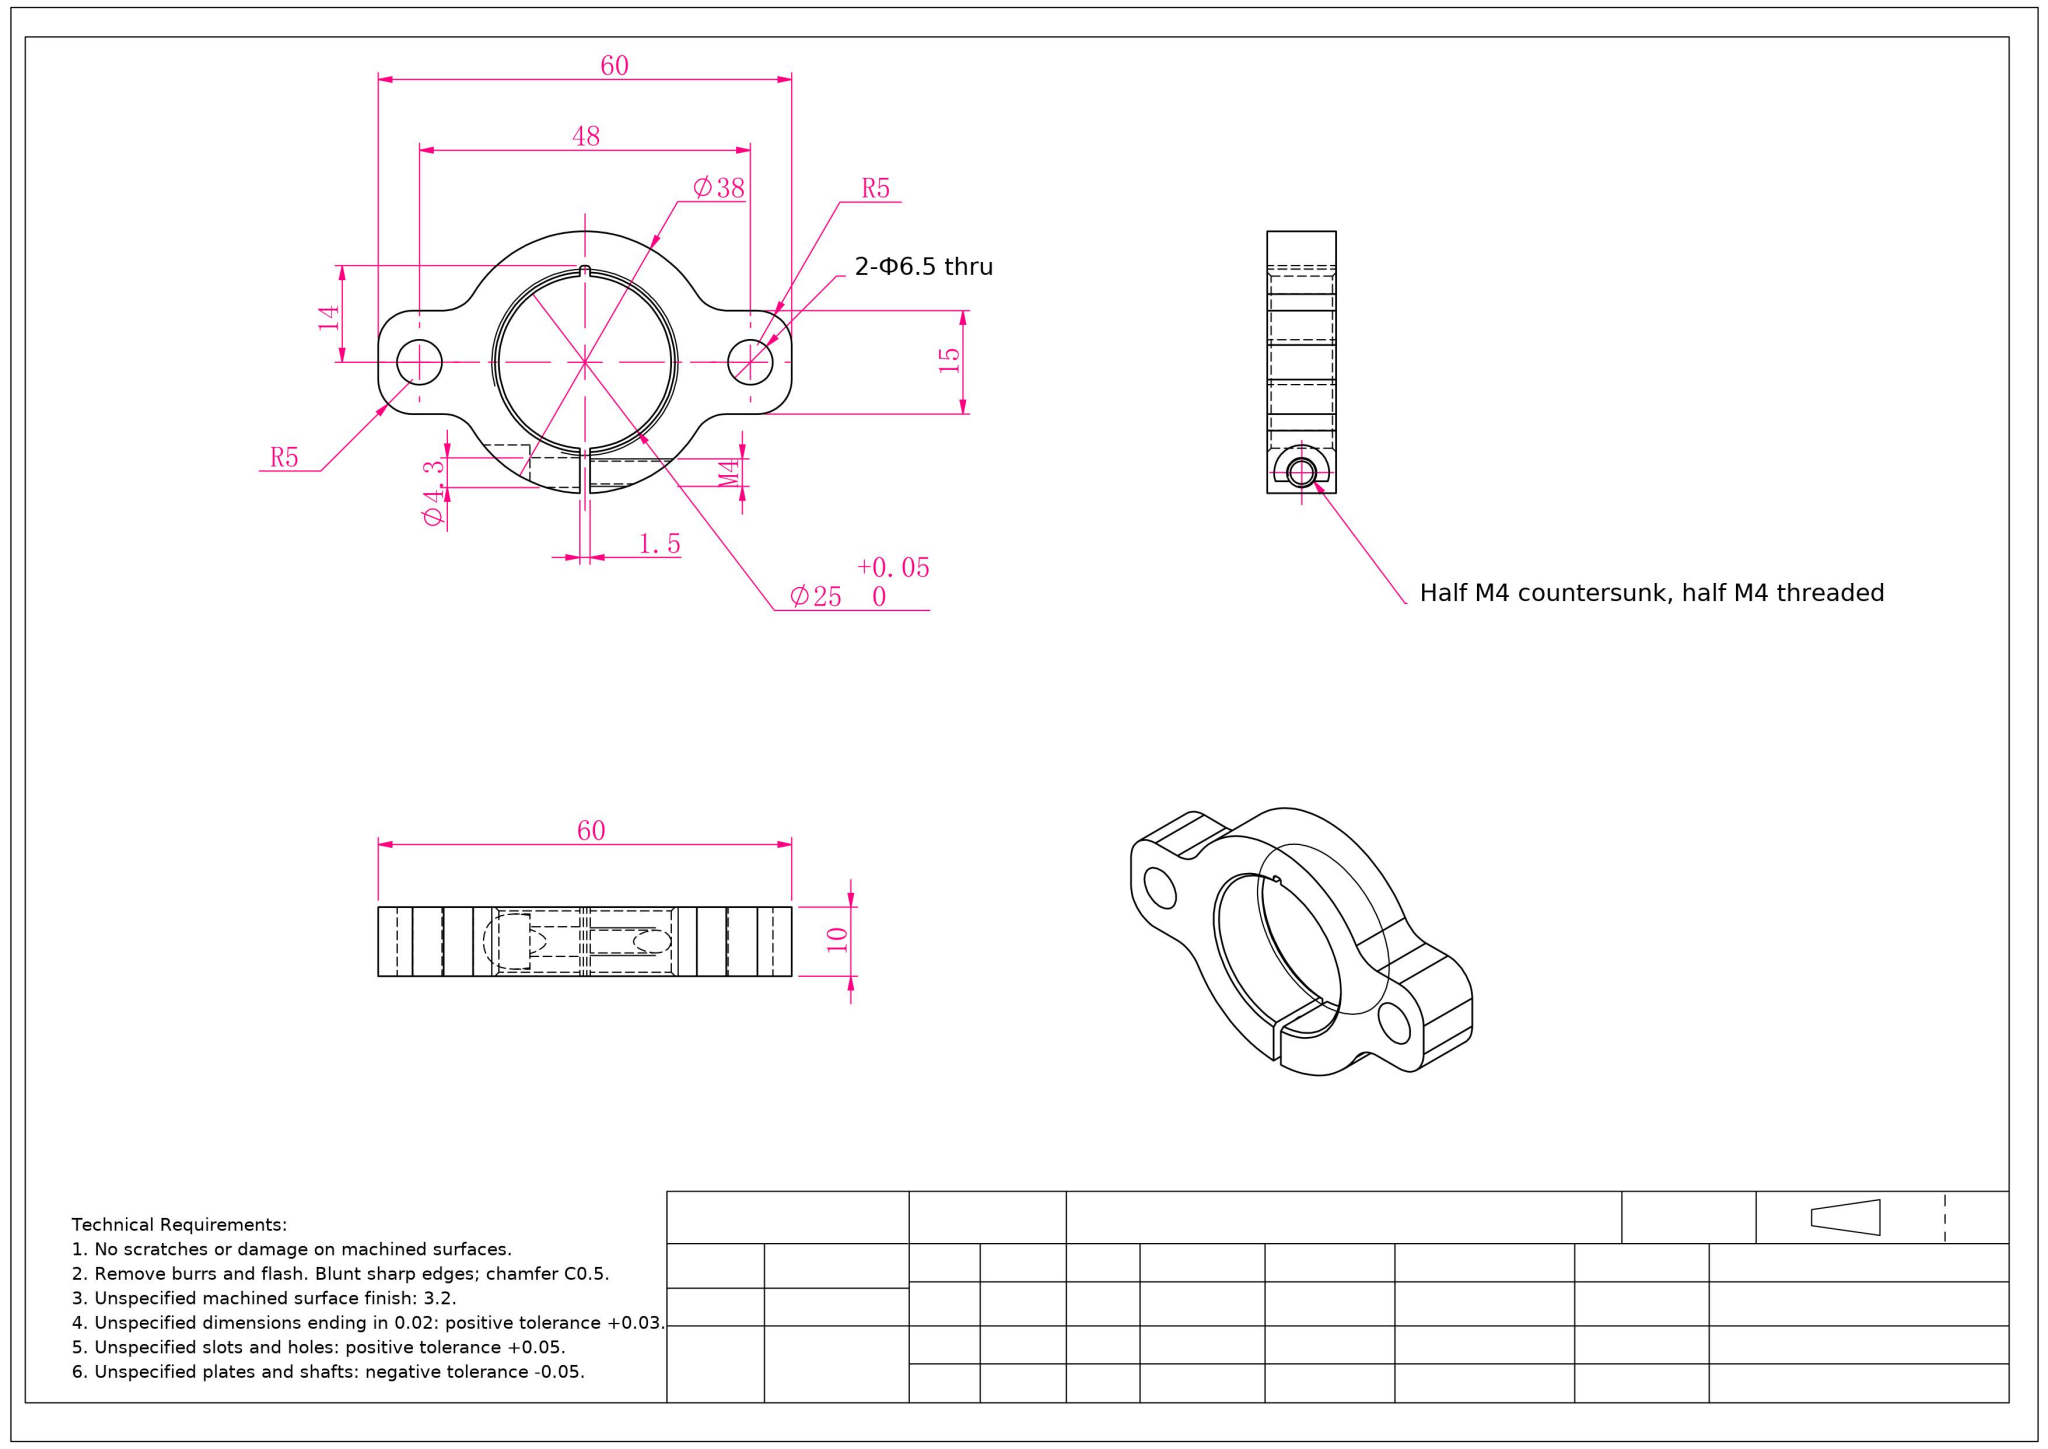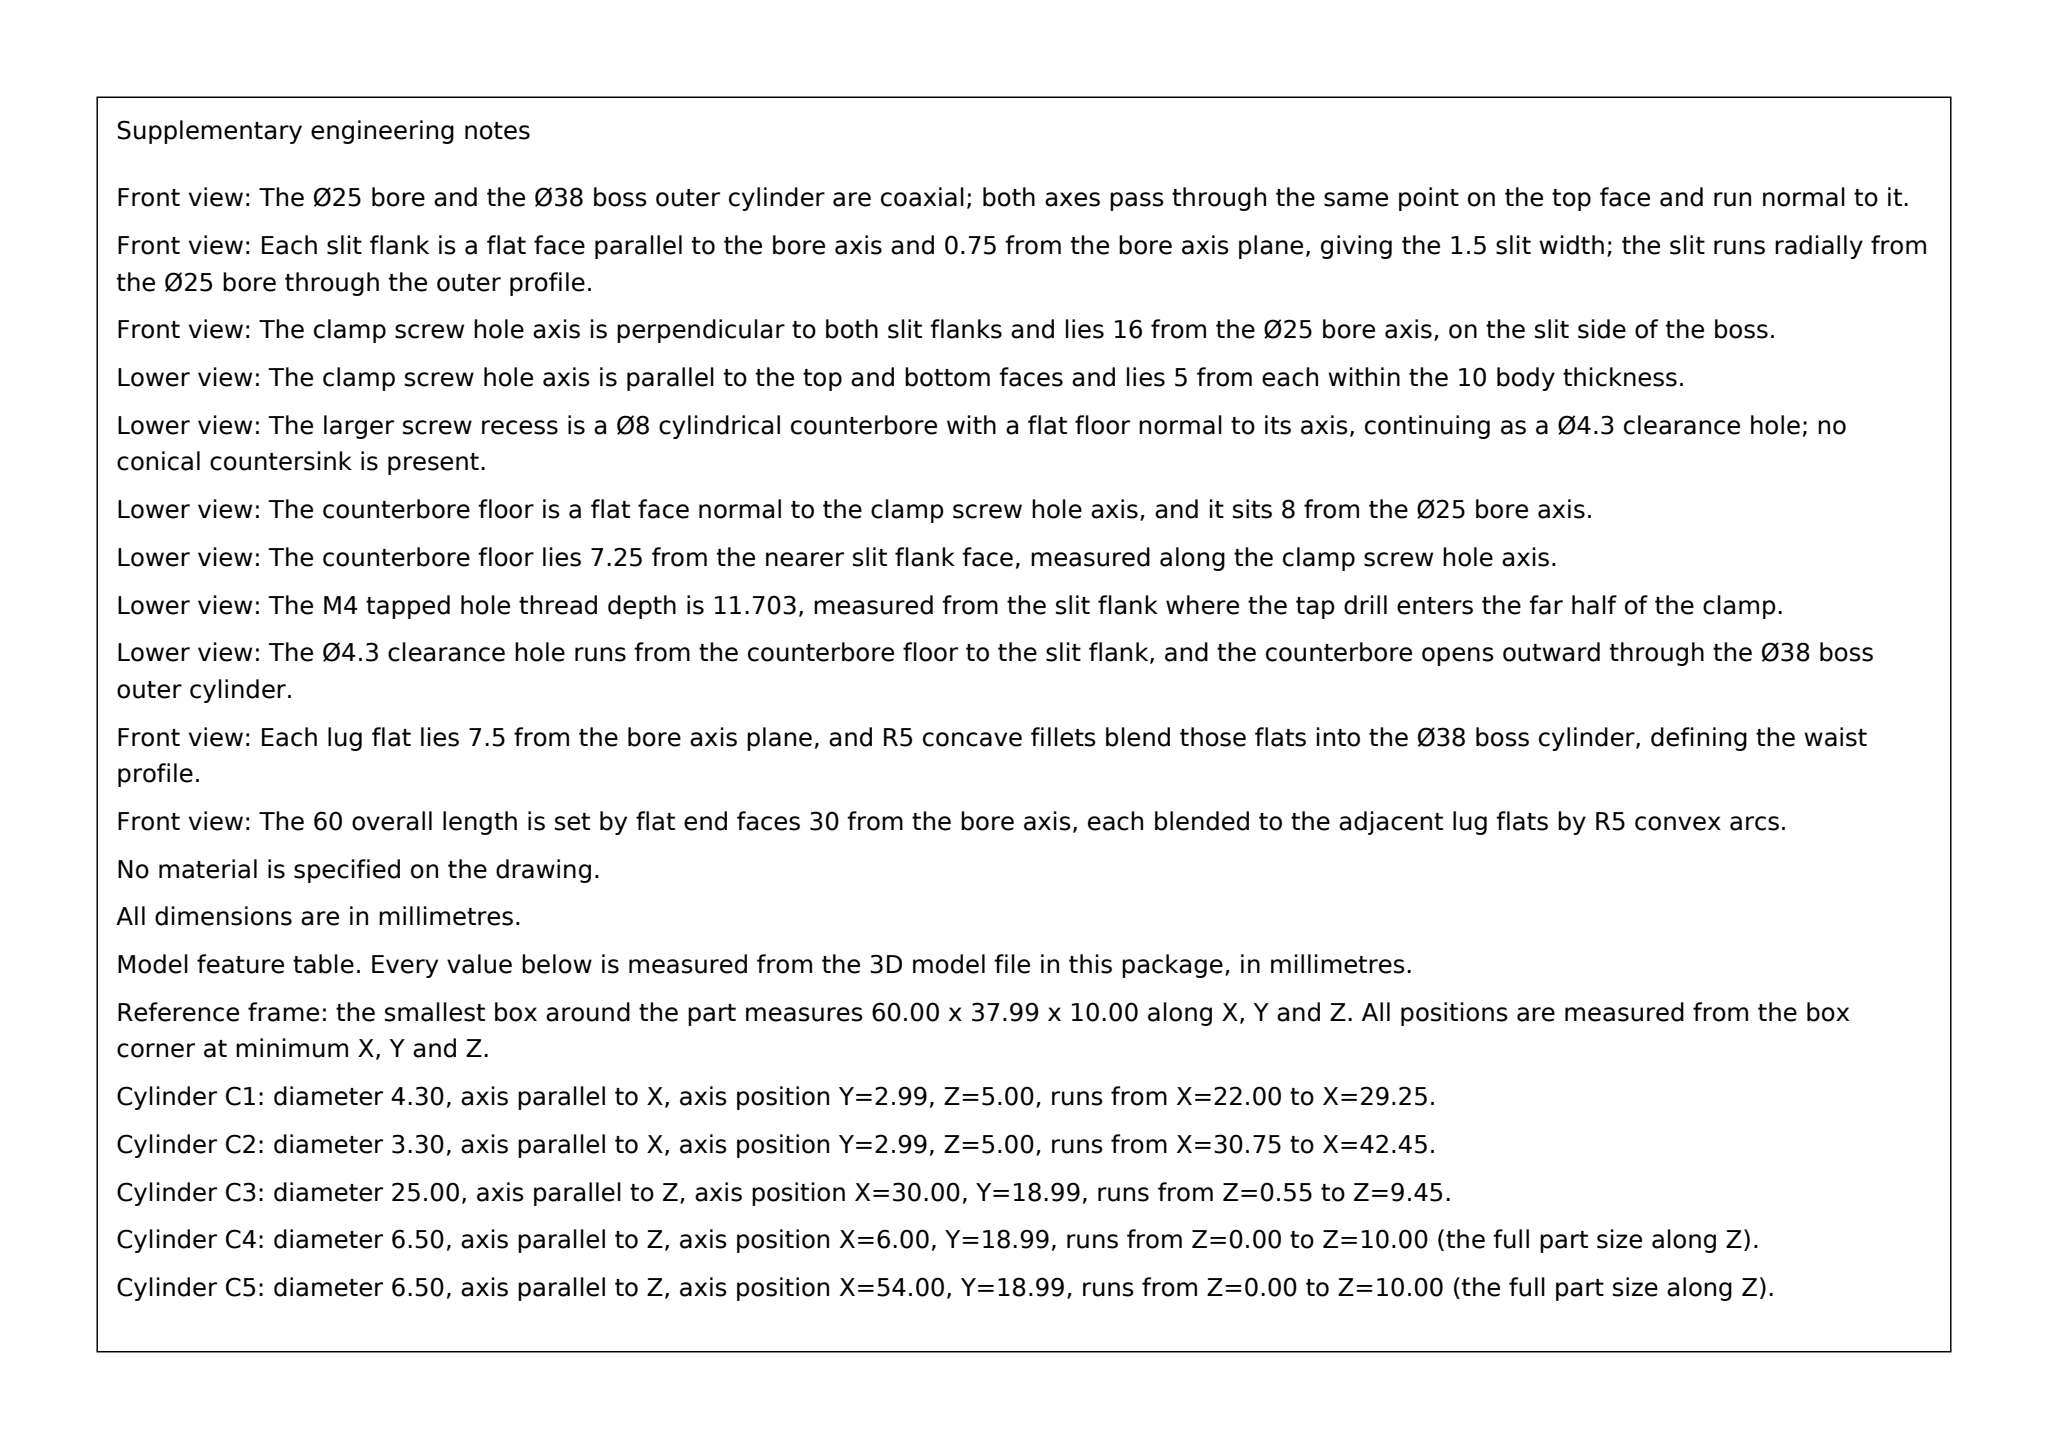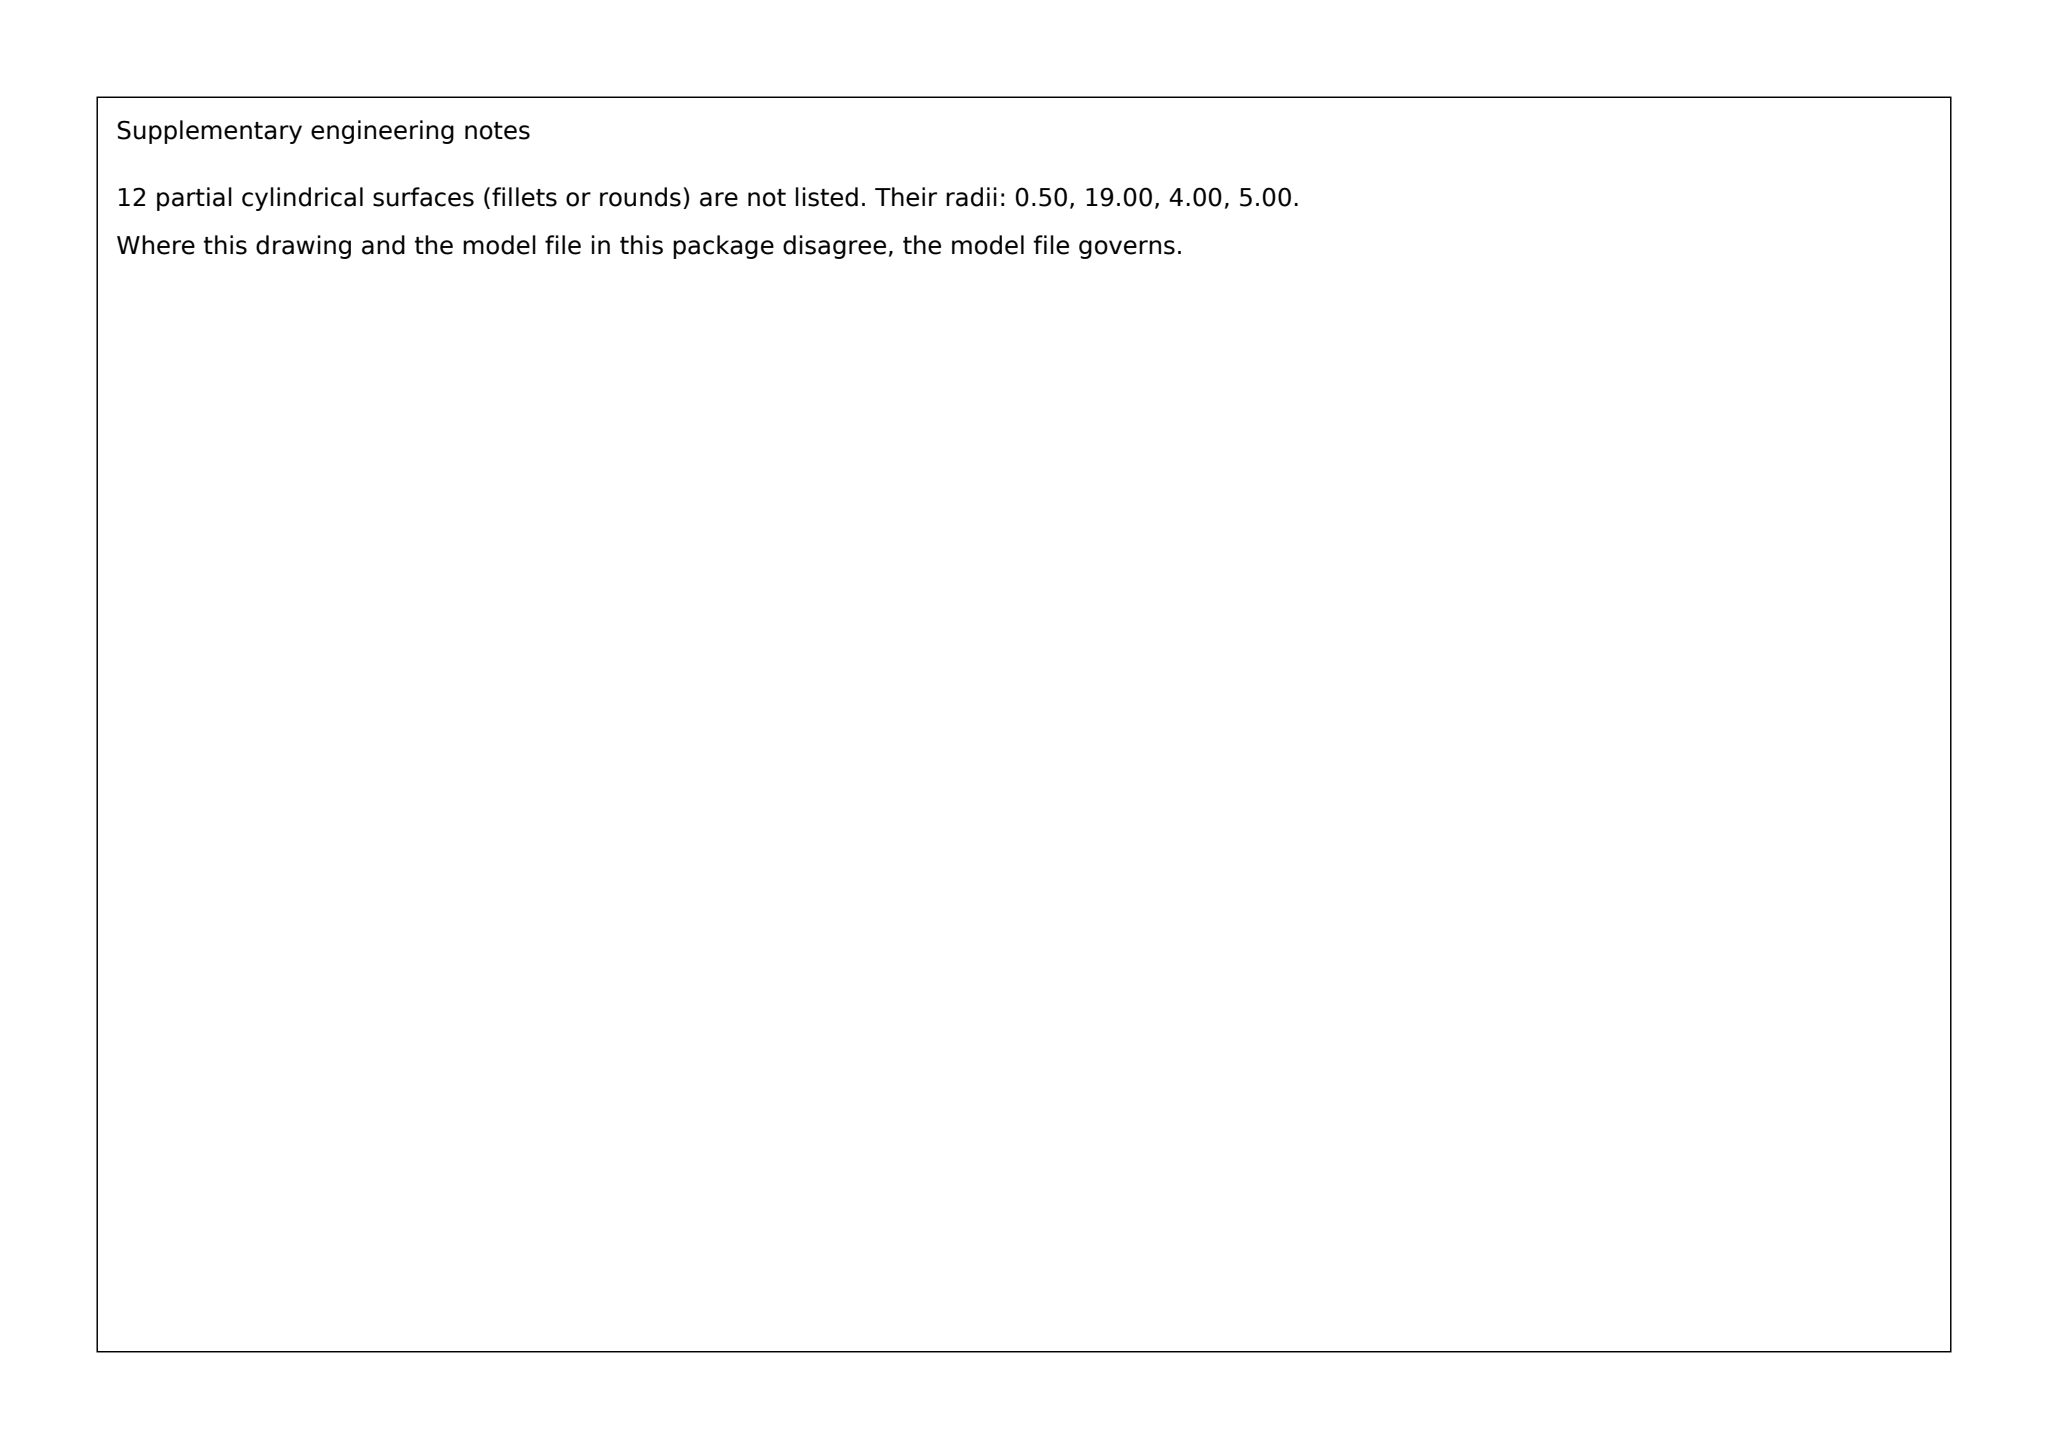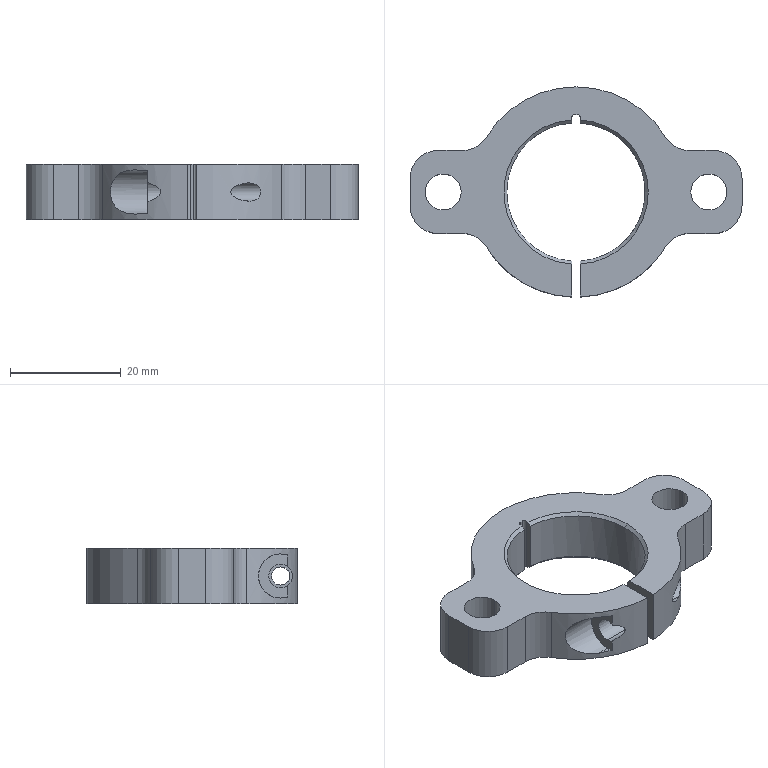Part | SolidWorks | mm | 1 solid | 47 faces | box 60 x 37.99 x 10 mm | volume 8615 mm3 | cylinder 27 | plane 14 | cone 6 | commonest cylinder face diameters 10 x8 6.5 x4 25 x3 8 x3 38 x3 4.3 x2 3.3 x2 1 x2
build123d program:
from build123d import *

# Parameters (mm, degrees)
SKETCH1_R                                       = 12.05
EXTRUDE1_DEPTH                                  = 10
SKETCH2_R                                       = 3.25
EXTRUDE2_DEPTH                                  = 37.892
EXTRUDE3_DEPTH                                  = 37.892
SKETCH4_W                                       = 1.65
SKETCH4_H                                       = 29.25
M4_HEX_SOCKET_HEAD_CAP_SCREW_HOLE_1_D           = 4.3
M4_HEX_SOCKET_HEAD_CAP_SCREW_HOLE_1_DEPTH       = 17.25
M4_HEX_SOCKET_HEAD_CAP_SCREW_HOLE_1_CBORE_D     = 8
M4_HEX_SOCKET_HEAD_CAP_SCREW_HOLE_1_CBORE_DEPTH = 10
FILLET1_R                                       = 5
CHAMFER1_SIZE                                   = 1
M27X2_0_TAPPED_HOLE1_D                          = 25


with BuildPart() as part:
    # Sketch1 → Extrude1 (new body)
    with BuildSketch(Plane.XY):
        with BuildLine():
            Line((-25, -7.5), (-17.457, -7.5))
            ThreePointArc((-17.457, -7.5), (0, -19), (17.457, -7.5))
            Line((17.457, -7.5), (25, -7.5))
            ThreePointArc((25, -7.5), (28.536, -6.036), (30, -2.5))
            Line((30, -2.5), (30, 2.5))
            ThreePointArc((30, 2.5), (28.536, 6.036), (25, 7.5))
            Line((25, 7.5), (17.457, 7.5))
            ThreePointArc((17.457, 7.5), (0, 19), (-17.457, 7.5))
            Line((-17.457, 7.5), (-25, 7.5))
            ThreePointArc((-25, 7.5), (-28.536, 6.036), (-30, 2.5))
            Line((-30, 2.5), (-30, -2.5))
            ThreePointArc((-30, -2.5), (-28.536, -6.036), (-25, -7.5))
        make_face()
        Circle(SKETCH1_R, mode=Mode.SUBTRACT)
    extrude(amount=EXTRUDE1_DEPTH)

    # Sketch2 → Extrude2 (cut, through all)
    with BuildSketch(Plane(origin=(0, 0, 0), x_dir=(-1, 0, 0), z_dir=(0, 0, -1))):
        with Locations((-24, 0)):
            Circle(SKETCH2_R)
        with Locations((24, 0)):
            Circle(SKETCH2_R)
    extrude(amount=-EXTRUDE2_DEPTH, mode=Mode.SUBTRACT)

    # Sketch3 → Extrude3 (cut, through all)
    with BuildSketch(Plane.XY.offset(10)):
        with BuildLine():
            Line((-0.25, 14), (0.25, 14))
            ThreePointArc((0.25, 14), (0.6036, 13.854), (0.75, 13.5))
            Line((0.75, 13.5), (0.75, -26.662))
            Line((0.75, -26.662), (-0.75, -26.662))
            Line((-0.75, -26.662), (-0.75, 13.5))
            ThreePointArc((-0.75, 13.5), (-0.6036, 13.854), (-0.25, 14))
        make_face()
    extrude(amount=-EXTRUDE3_DEPTH, mode=Mode.SUBTRACT)

    # Sketch4 → M4 Tapped Hole1 (revolve, cut)
    with BuildSketch(Plane(origin=(0.75, -16, 5), x_dir=(0, 0, 1), z_dir=(0, 1, 0))):
        with Locations((0.825, 14.625)):
            Rectangle(SKETCH4_W, SKETCH4_H)
    revolve(axis=Axis((-5.6, -16, 5), (1, 0, 0)), mode=Mode.SUBTRACT)

    # M4 Hex Socket Head Cap Screw Hole 1
    with Locations(Plane(origin=(-18, 0, 0), x_dir=(0, 0, -1), z_dir=(-1, 0, 0))):
        with Locations((-5, 16)):
            CounterBoreHole(M4_HEX_SOCKET_HEAD_CAP_SCREW_HOLE_1_D / 2, M4_HEX_SOCKET_HEAD_CAP_SCREW_HOLE_1_CBORE_D / 2, M4_HEX_SOCKET_HEAD_CAP_SCREW_HOLE_1_CBORE_DEPTH, depth=M4_HEX_SOCKET_HEAD_CAP_SCREW_HOLE_1_DEPTH)

    # Fillet1
    fillet1_edges = [part.edges().sort_by_distance(p)[0] for p in [
        (-17.457, -7.5, 5),
        (-17.457, 7.5, 5),
        (17.457, 7.5, 5),
        (17.457, -7.5, 5),
    ]]
    fillet(fillet1_edges, radius=FILLET1_R)

    # Chamfer1
    chamfer1_edges = [part.edges().sort_by_distance(p)[0] for p in [
        (-12.05, 0, 10),
        (12.05, 0, 10),
        (-12.05, 0, 0),
        (12.05, 0, 0),
    ]]
    chamfer(chamfer1_edges, length=CHAMFER1_SIZE)

    # M27x2.0 Tapped Hole1 (through all)
    with Locations(Plane(origin=(0, 0, 0), x_dir=(-1, 0, 0), z_dir=(0, 0, -1))):
        with Locations((0, 0)):
            Hole(M27X2_0_TAPPED_HOLE1_D / 2)


solid = part.part